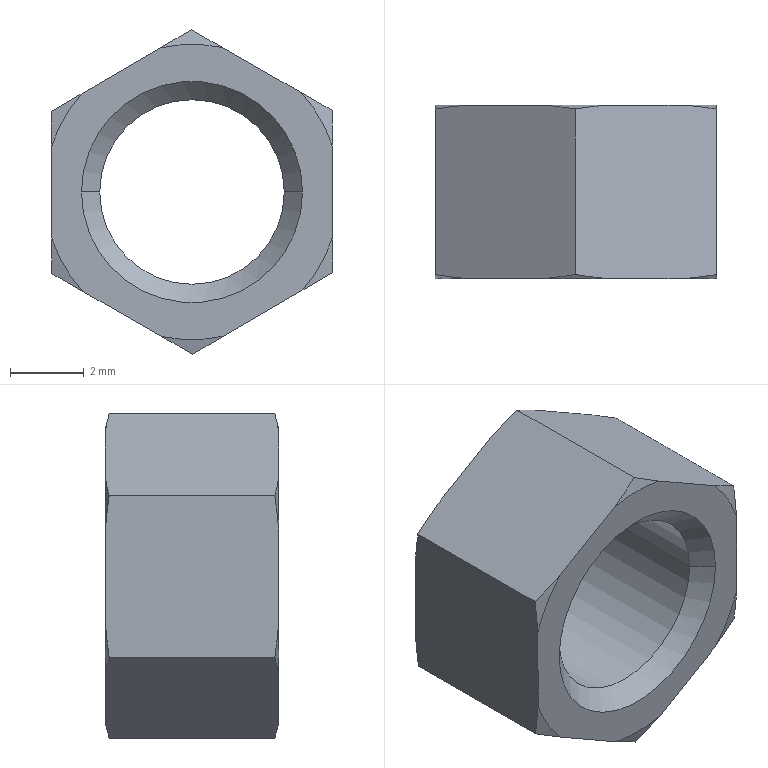Component | SolidWorks | GB_T6170-2000Type1HexNutGradeAAndBM5-1 | 1 solid | 26 faces | volume 139 mm3 | cone 16 | plane 8 | cylinder 2 | commonest cylinder face diameters 5 x2 | material AISI 321 Annealed Stainless Steel (SS)